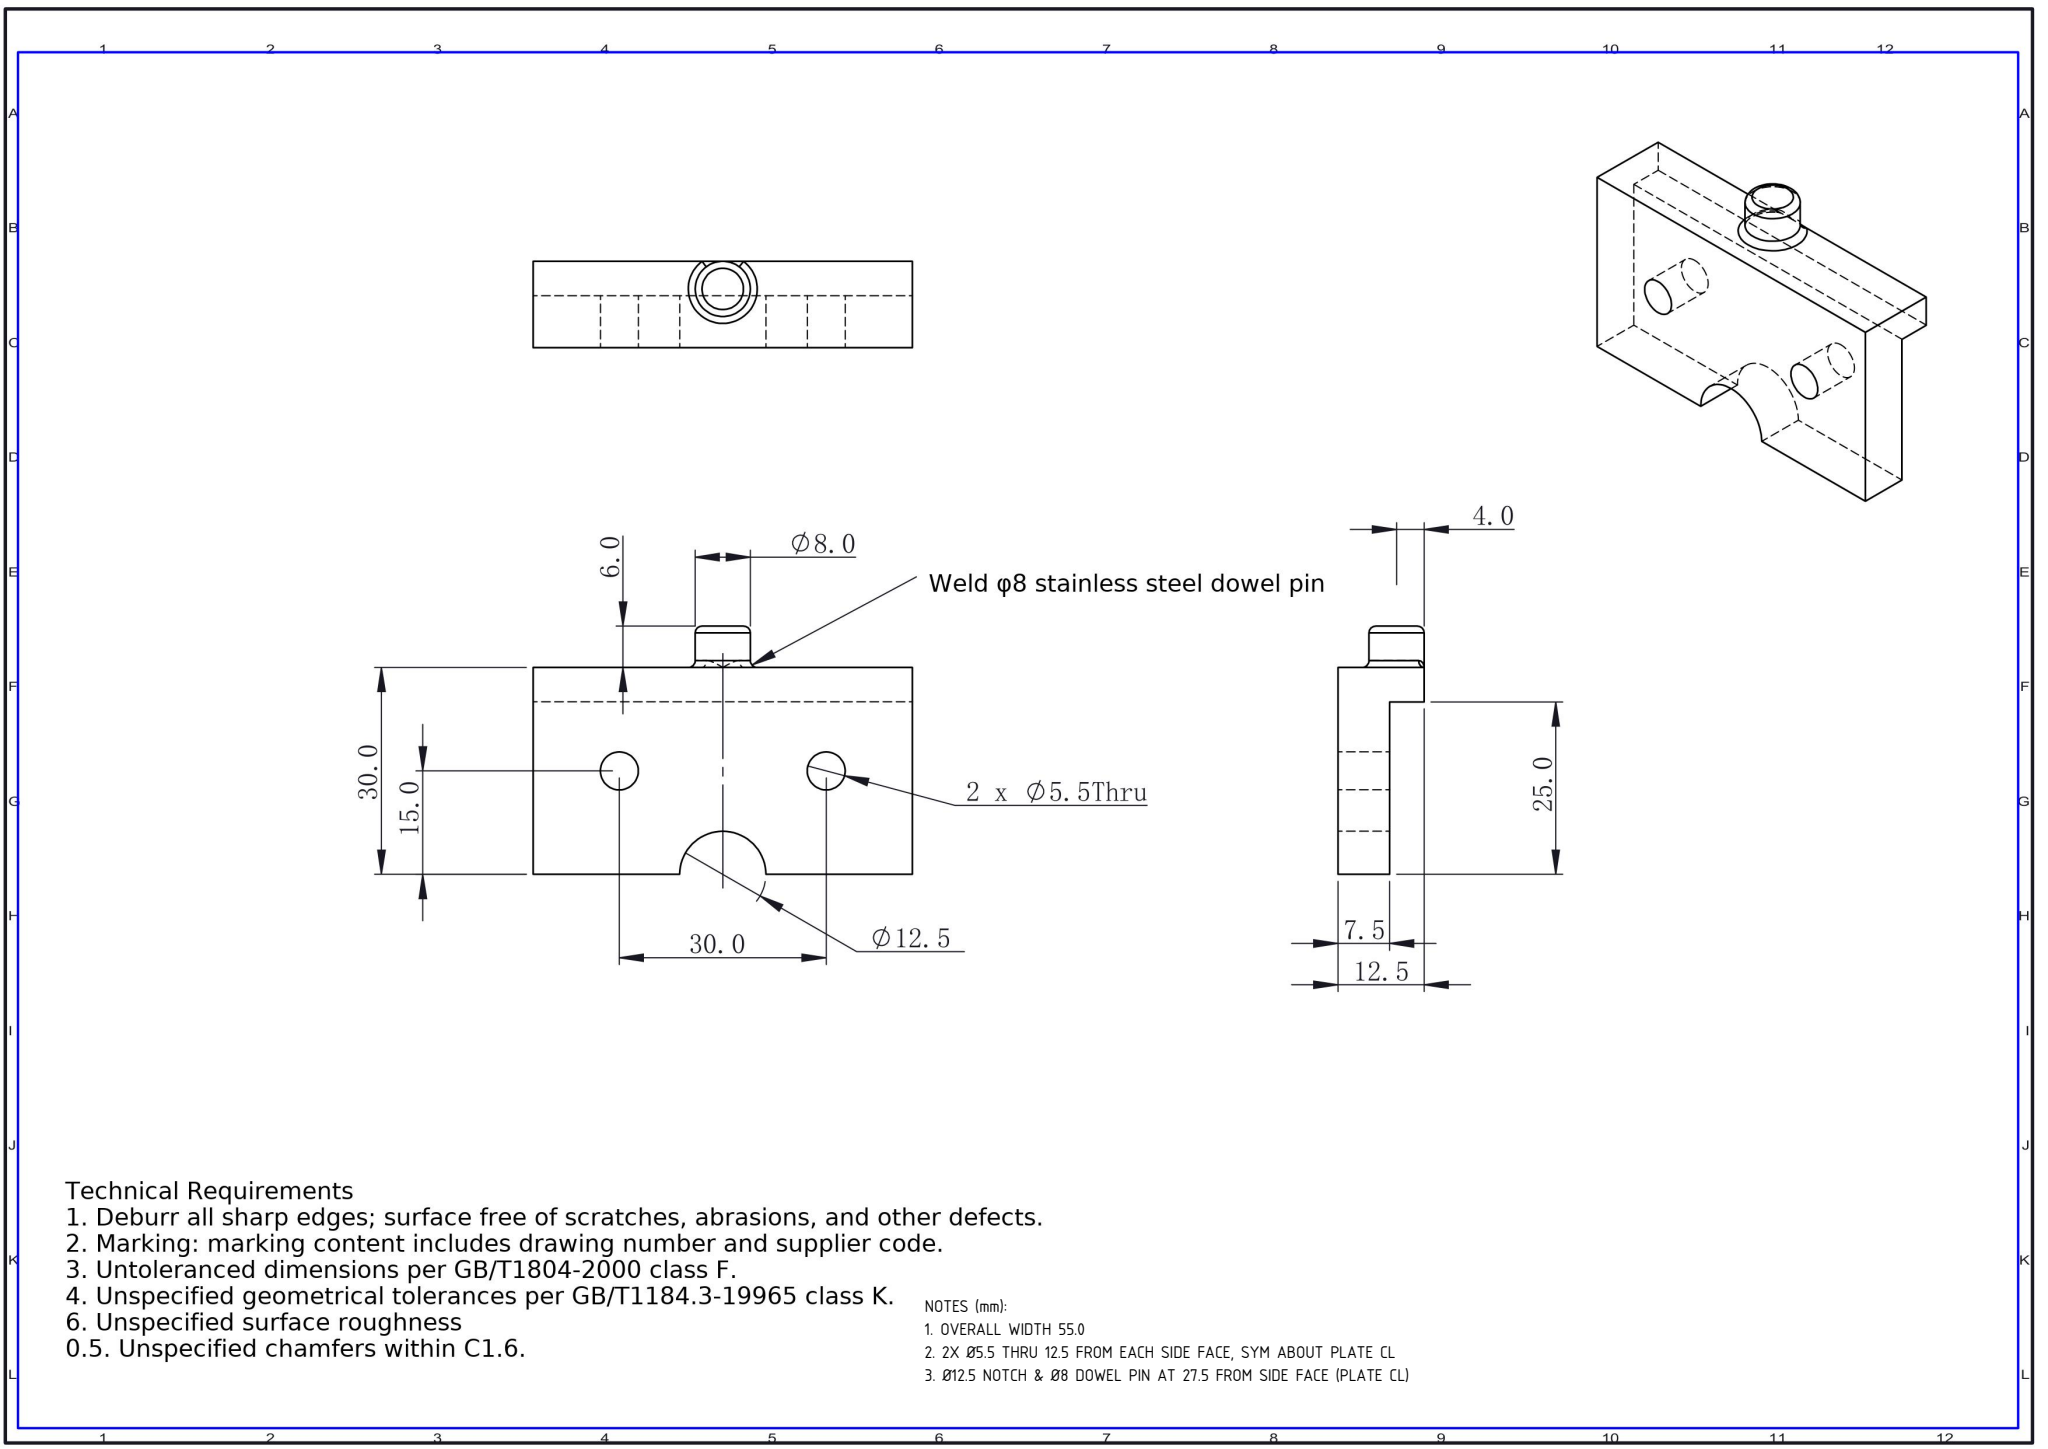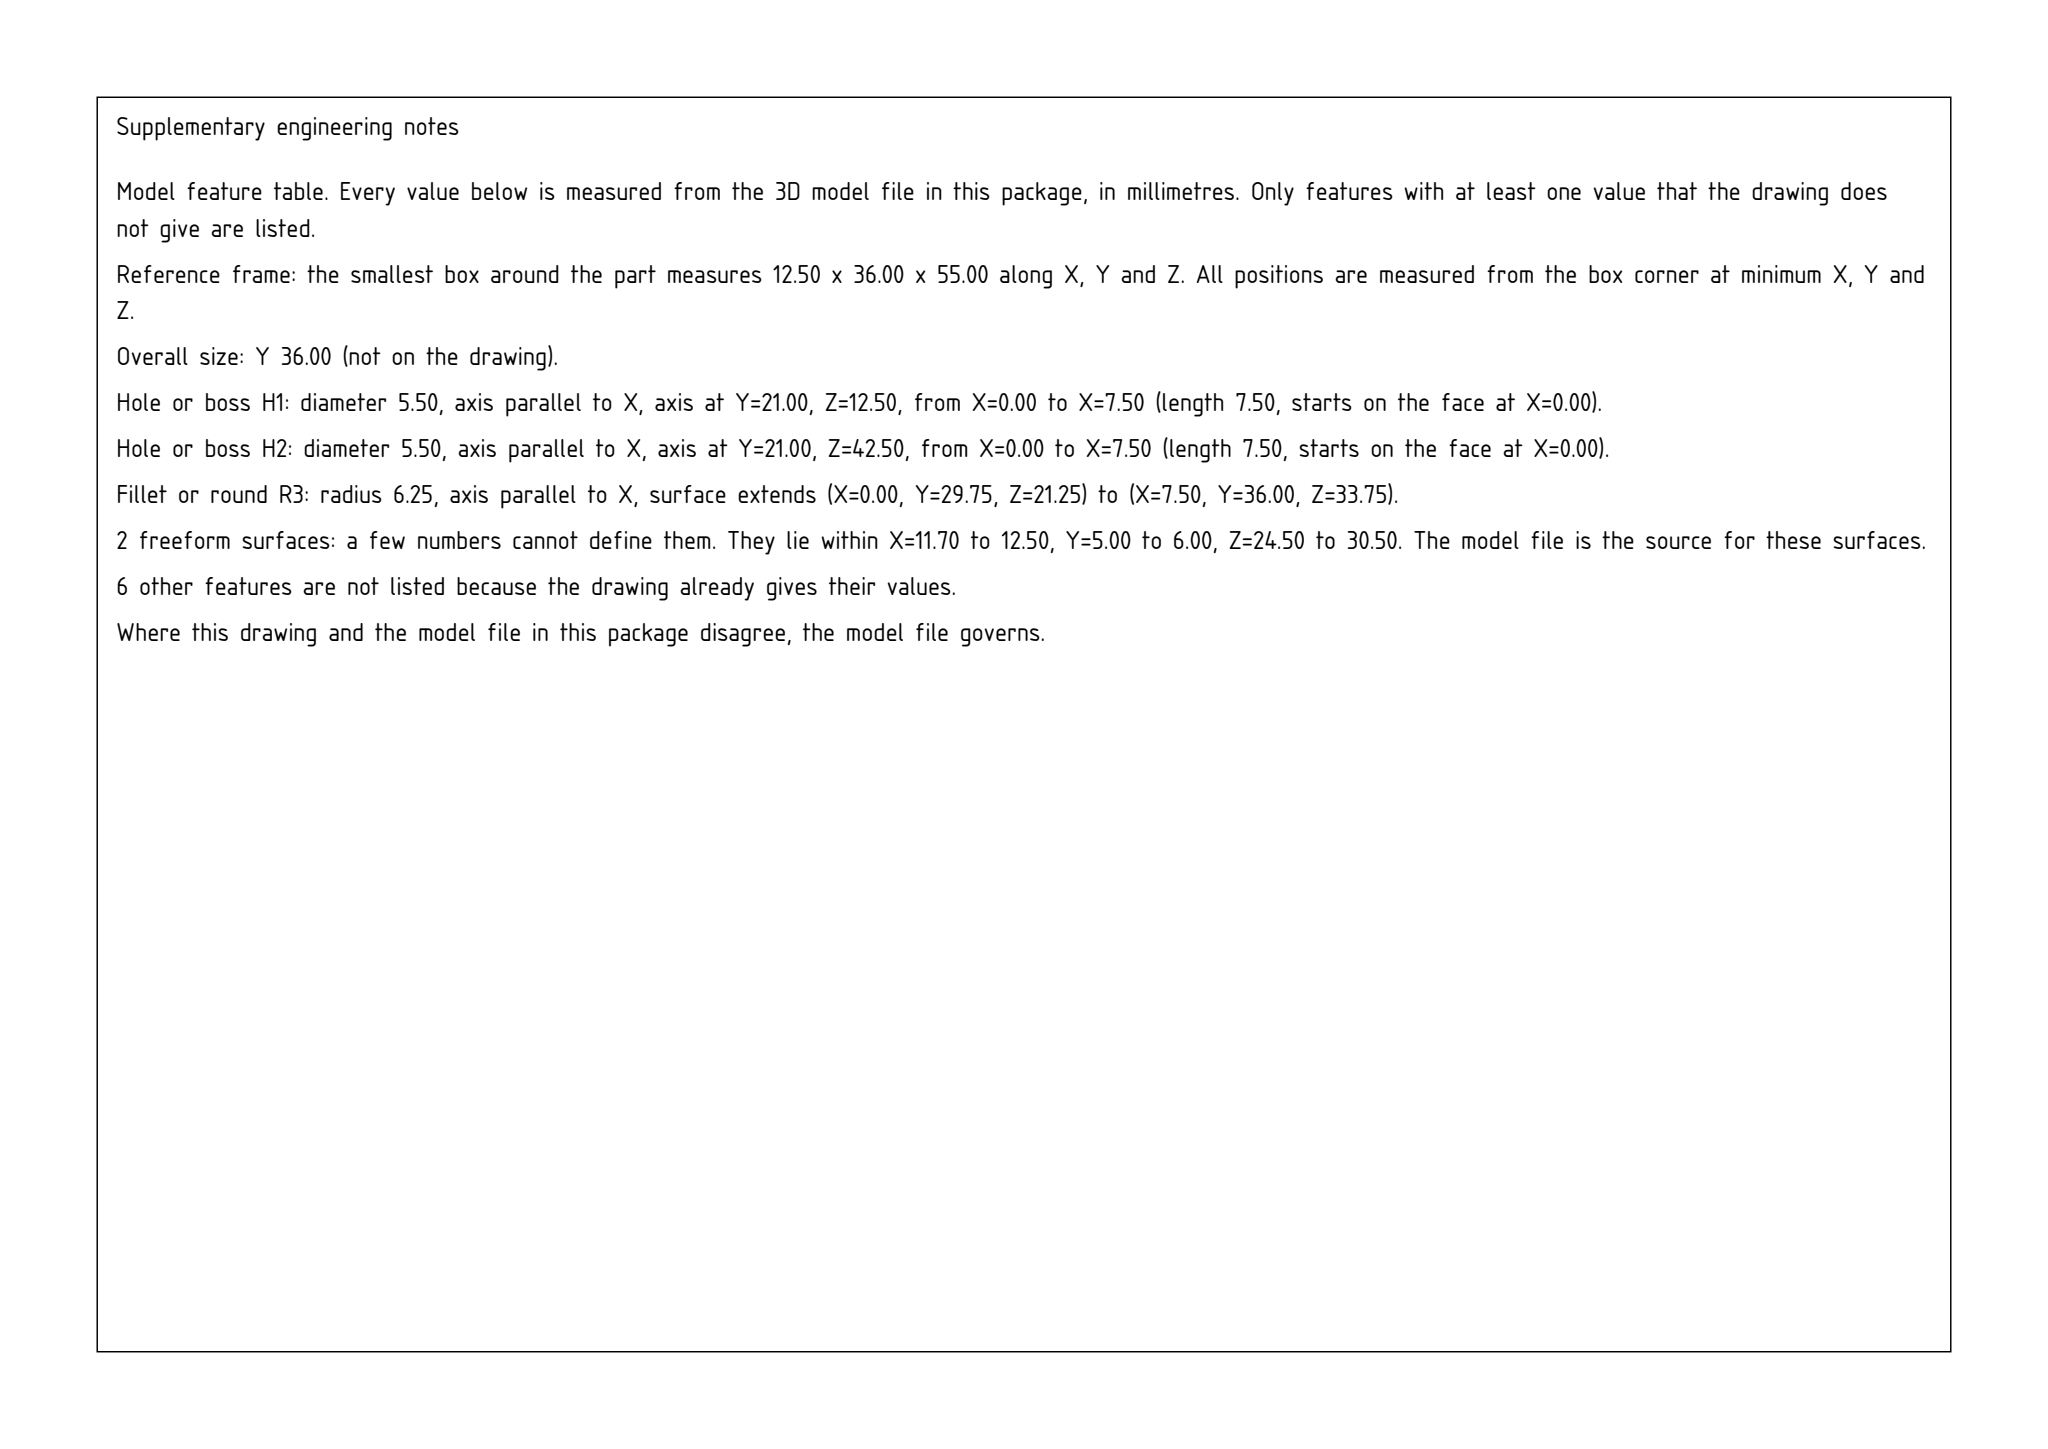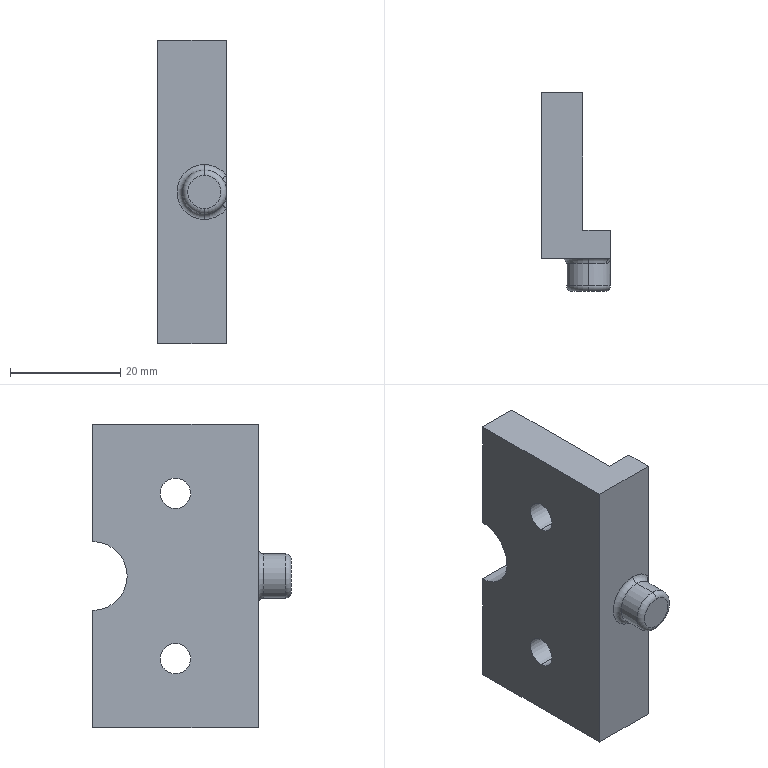Part | SolidWorks | mm | 1 solid | 25 faces | box 12.5 x 36 x 55 mm | volume 13235 mm3 | plane 10 | cylinder 8 | torus 5 | spline 2 | commonest cylinder face diameters 5.5 x4 8 x2 12.5 x2
Drawing notes:
OVERALL WIDTH 55.0 | from the solid: bbox z = 55.0 (planes z=0 and z=55)
2X Ø5.5 THRU 12.5 FROM EACH SIDE FACE, SYM ABOUT PLATE CL | from the solid: cyl Ø5.5 at z=12.5 and z=42.5, width 55.0
Ø12.5 NOTCH & Ø8 DOWEL PIN AT 27.5 FROM SIDE FACE (PLATE CL) | from the solid: Ø12.5 and Ø8 axes at z=27.5 = 55.0/2
STEP:
#1=CARTESIAN_POINT('',(8.5,-35.,31.5));
#2=VERTEX_POINT('',#1);
#3=CARTESIAN_POINT('',(8.5,-35.,23.5));
#4=VERTEX_POINT('',#3);
#5=CARTESIAN_POINT('',(8.5,-35.,27.5));
#6=DIRECTION('',(0.,1.,0.));
#7=DIRECTION('',(0.,0.,-1.));
#8=AXIS2_PLACEMENT_3D('',#5,#6,#7);
#9=CIRCLE('',#8,4.);
#10=EDGE_CURVE('',#2,#4,#9,.T.);
#11=ORIENTED_EDGE('',*,*,#10,.F.);
#12=CARTESIAN_POINT('',(8.5,-36.,30.5));
#13=VERTEX_POINT('',#12);
#14=CARTESIAN_POINT('',(8.5,-35.,30.5));
#15=DIRECTION('',(1.,0.,-0.));
#16=DIRECTION('',(0.,0.,-1.));
#17=AXIS2_PLACEMENT_3D('',#14,#15,#16);
#18=CIRCLE('',#17,1.);
#19=EDGE_CURVE('',#2,#13,#18,.T.);
#20=ORIENTED_EDGE('',*,*,#19,.T.);
#21=CARTESIAN_POINT('',(8.5,-36.,24.5));
#22=VERTEX_POINT('',#21);
#23=CARTESIAN_POINT('',(8.5,-36.,27.5));
#24=DIRECTION('',(0.,-1.,0.));
#25=DIRECTION('',(0.,0.,-1.));
#26=AXIS2_PLACEMENT_3D('',#23,#24,#25);
#27=CIRCLE('',#26,3.);
#28=EDGE_CURVE('',#22,#13,#27,.T.);
#29=ORIENTED_EDGE('',*,*,#28,.F.);
#30=CARTESIAN_POINT('',(8.5,-35.,24.5));
#31=DIRECTION('',(-1.,0.,0.));
#32=DIRECTION('',(0.,0.,1.));
#33=AXIS2_PLACEMENT_3D('',#30,#31,#32);
#34=CIRCLE('',#33,1.);
#35=EDGE_CURVE('',#4,#22,#34,.T.);
#36=ORIENTED_EDGE('',*,*,#35,.F.);
#37=EDGE_LOOP('',(#11,#20,#29,#36));
#38=FACE_OUTER_BOUND('',#37,.T.);
#39=CARTESIAN_POINT('',(8.5,-35.,27.5));
#40=DIRECTION('',(0.,-1.,0.));
#41=DIRECTION('',(0.,0.,-1.));
#42=AXIS2_PLACEMENT_3D('',#39,#40,#41);
#43=TOROIDAL_SURFACE('',#42,3.,1.);
#44=ADVANCED_FACE('',(#38),#43,.T.);
#45=CARTESIAN_POINT('',(8.5,-30.,22.5));
#46=VERTEX_POINT('',#45);
#47=CARTESIAN_POINT('',(8.5,-30.,32.5));
#48=VERTEX_POINT('',#47);
#49=CARTESIAN_POINT('',(8.5,-30.,27.5));
#50=DIRECTION('',(0.,1.,0.));
#51=DIRECTION('',(0.,0.,1.));
#52=AXIS2_PLACEMENT_3D('',#49,#50,#51);
#53=CIRCLE('',#52,5.);
#54=EDGE_CURVE('',#46,#48,#53,.T.);
#55=ORIENTED_EDGE('',*,*,#54,.F.);
#56=CARTESIAN_POINT('',(8.5,-31.,23.5));
#57=VERTEX_POINT('',#56);
#58=CARTESIAN_POINT('',(8.5,-31.,22.5));
#59=DIRECTION('',(1.,0.,0.));
#60=DIRECTION('',(0.,0.,-1.));
#61=AXIS2_PLACEMENT_3D('',#58,#59,#60);
#62=CIRCLE('',#61,1.);
#63=EDGE_CURVE('',#46,#57,#62,.T.);
#64=ORIENTED_EDGE('',*,*,#63,.T.);
#65=CARTESIAN_POINT('',(8.5,-31.,31.5));
#66=VERTEX_POINT('',#65);
#67=CARTESIAN_POINT('',(8.5,-31.,27.5));
#68=DIRECTION('',(0.,-1.,0.));
#69=DIRECTION('',(0.,0.,1.));
#70=AXIS2_PLACEMENT_3D('',#67,#68,#69);
#71=CIRCLE('',#70,4.);
#72=EDGE_CURVE('',#66,#57,#71,.T.);
#73=ORIENTED_EDGE('',*,*,#72,.F.);
#74=CARTESIAN_POINT('',(8.5,-31.,32.5));
#75=DIRECTION('',(-1.,0.,0.));
#76=DIRECTION('',(0.,0.,1.));
#77=AXIS2_PLACEMENT_3D('',#74,#75,#76);
#78=CIRCLE('',#77,1.);
#79=EDGE_CURVE('',#48,#66,#78,.T.);
#80=ORIENTED_EDGE('',*,*,#79,.F.);
#81=EDGE_LOOP('',(#55,#64,#73,#80));
#82=FACE_OUTER_BOUND('',#81,.T.);
#83=CARTESIAN_POINT('',(8.5,-31.,27.5));
#84=DIRECTION('',(0.,1.,0.));
#85=DIRECTION('',(0.,0.,1.));
#86=AXIS2_PLACEMENT_3D('',#83,#84,#85);
#87=TOROIDAL_SURFACE('',#86,5.,1.);
#88=ADVANCED_FACE('',(#82),#87,.F.);
#89=CARTESIAN_POINT('',(12.5,-30.,30.5));
#90=VERTEX_POINT('',#89);
#91=CARTESIAN_POINT('',(8.5,-30.,27.5));
#92=DIRECTION('',(0.,1.,0.));
#93=DIRECTION('',(0.,0.,1.));
#94=AXIS2_PLACEMENT_3D('',#91,#92,#93);
#95=CIRCLE('',#94,5.);
#96=EDGE_CURVE('',#48,#90,#95,.T.);
#97=ORIENTED_EDGE('',*,*,#96,.F.);
#98=ORIENTED_EDGE('',*,*,#79,.T.);
#99=CARTESIAN_POINT('',(11.7,-31.,29.9));
#100=VERTEX_POINT('',#99);
#101=CARTESIAN_POINT('',(8.5,-31.,27.5));
#102=DIRECTION('',(0.,-1.,0.));
#103=DIRECTION('',(0.,0.,1.));
#104=AXIS2_PLACEMENT_3D('',#101,#102,#103);
#105=CIRCLE('',#104,4.);
#106=EDGE_CURVE('',#100,#66,#105,.T.);
#107=ORIENTED_EDGE('',*,*,#106,.F.);
#108=CARTESIAN_POINT('',(12.5,-31.,30.5));
#109=DIRECTION('',(-0.6,0.,0.8));
#110=DIRECTION('',(0.8,0.,0.6));
#111=AXIS2_PLACEMENT_3D('',#108,#109,#110);
#112=CIRCLE('',#111,1.);
#113=EDGE_CURVE('',#90,#100,#112,.T.);
#114=ORIENTED_EDGE('',*,*,#113,.F.);
#115=EDGE_LOOP('',(#97,#98,#107,#114));
#116=FACE_OUTER_BOUND('',#115,.T.);
#117=CARTESIAN_POINT('',(8.5,-31.,27.5));
#118=DIRECTION('',(0.,1.,0.));
#119=DIRECTION('',(0.,0.,1.));
#120=AXIS2_PLACEMENT_3D('',#117,#118,#119);
#121=TOROIDAL_SURFACE('',#120,5.,1.);
#122=ADVANCED_FACE('',(#116),#121,.F.);
#123=ORIENTED_EDGE('',*,*,#10,.T.);
#124=CARTESIAN_POINT('',(8.5,-36.,23.5));
#125=DIRECTION('',(0.,1.,0.));
#126=VECTOR('',#125,1000.);
#127=LINE('',#124,#126);
#128=EDGE_CURVE('',#4,#57,#127,.T.);
#129=ORIENTED_EDGE('',*,*,#128,.T.);
#130=CARTESIAN_POINT('',(11.7,-31.,25.1));
#131=VERTEX_POINT('',#130);
#132=CARTESIAN_POINT('',(8.5,-31.,27.5));
#133=DIRECTION('',(0.,-1.,0.));
#134=DIRECTION('',(0.,0.,1.));
#135=AXIS2_PLACEMENT_3D('',#132,#133,#134);
#136=CIRCLE('',#135,4.);
#137=EDGE_CURVE('',#57,#131,#136,.T.);
#138=ORIENTED_EDGE('',*,*,#137,.T.);
#139=CARTESIAN_POINT('',(12.5,-30.,27.5));
#140=VERTEX_POINT('',#139);
#141=CARTESIAN_POINT('',(11.7,-31.,25.1));
#142=CARTESIAN_POINT('',(11.842,-31.,25.289));
#143=CARTESIAN_POINT('',(11.961,-30.956,25.482));
#144=CARTESIAN_POINT('',(12.165,-30.826,25.882));
#145=CARTESIAN_POINT('',(12.247,-30.741,26.083));
#146=CARTESIAN_POINT('',(12.375,-30.551,26.485));
#147=CARTESIAN_POINT('',(12.422,-30.447,26.686));
#148=CARTESIAN_POINT('',(12.485,-30.227,27.093));
#149=CARTESIAN_POINT('',(12.5,-30.113,27.298));
#150=CARTESIAN_POINT('',(12.5,-30.,27.5));
#151=B_SPLINE_CURVE_WITH_KNOTS('',3,(#141,#142,#143,#144,#145,#146,#147,#148,#149,#150),.UNSPECIFIED.,.F.,.F.,(4,2,2,2,4),(0.,0.0006946,0.001389,0.002084,0.002779),.UNSPECIFIED.);
#152=EDGE_CURVE('',#131,#140,#151,.T.);
#153=ORIENTED_EDGE('',*,*,#152,.T.);
#154=CARTESIAN_POINT('',(12.5,-30.,27.5));
#155=CARTESIAN_POINT('',(12.5,-30.227,27.907));
#156=CARTESIAN_POINT('',(12.439,-30.457,28.315));
#157=CARTESIAN_POINT('',(12.247,-30.741,28.917));
#158=CARTESIAN_POINT('',(12.165,-30.826,29.118));
#159=CARTESIAN_POINT('',(11.961,-30.956,29.518));
#160=CARTESIAN_POINT('',(11.842,-31.,29.711));
#161=CARTESIAN_POINT('',(11.7,-31.,29.9));
#162=B_SPLINE_CURVE_WITH_KNOTS('',3,(#154,#155,#156,#157,#158,#159,#160,#161),.UNSPECIFIED.,.F.,.F.,(4,2,2,4),(-0.00001266,0.001384,0.002083,0.002782),.UNSPECIFIED.);
#163=EDGE_CURVE('',#140,#100,#162,.T.);
#164=ORIENTED_EDGE('',*,*,#163,.T.);
#165=ORIENTED_EDGE('',*,*,#106,.T.);
#166=CARTESIAN_POINT('',(8.5,-36.,31.5));
#167=DIRECTION('',(0.,1.,0.));
#168=VECTOR('',#167,1000.);
#169=LINE('',#166,#168);
#170=EDGE_CURVE('',#2,#66,#169,.T.);
#171=ORIENTED_EDGE('',*,*,#170,.F.);
#172=EDGE_LOOP('',(#123,#129,#138,#153,#164,#165,#171));
#173=FACE_OUTER_BOUND('',#172,.T.);
#174=CARTESIAN_POINT('',(8.5,-36.,27.5));
#175=DIRECTION('',(0.,1.,0.));
#176=DIRECTION('',(0.,0.,1.));
#177=AXIS2_PLACEMENT_3D('',#174,#175,#176);
#178=CYLINDRICAL_SURFACE('',#177,4.);
#179=ADVANCED_FACE('',(#173),#178,.T.);
#180=CARTESIAN_POINT('',(7.5,-15.,9.75));
#181=VERTEX_POINT('',#180);
#182=CARTESIAN_POINT('',(7.5,-15.,15.25));
#183=VERTEX_POINT('',#182);
#184=CARTESIAN_POINT('',(7.5,-15.,12.5));
#185=DIRECTION('',(-1.,-0.,0.));
#186=DIRECTION('',(0.,-1.,0.));
#187=AXIS2_PLACEMENT_3D('',#184,#185,#186);
#188=CIRCLE('',#187,2.75);
#189=EDGE_CURVE('',#181,#183,#188,.T.);
#190=ORIENTED_EDGE('',*,*,#189,.F.);
#191=CARTESIAN_POINT('',(0.,-15.,9.75));
#192=VERTEX_POINT('',#191);
#193=CARTESIAN_POINT('',(0.,-15.,9.75));
#194=DIRECTION('',(-1.,0.,0.));
#195=VECTOR('',#194,1000.);
#196=LINE('',#193,#195);
#197=EDGE_CURVE('',#181,#192,#196,.T.);
#198=ORIENTED_EDGE('',*,*,#197,.T.);
#199=CARTESIAN_POINT('',(0.,-15.,15.25));
#200=VERTEX_POINT('',#199);
#201=CARTESIAN_POINT('',(0.,-15.,12.5));
#202=DIRECTION('',(-1.,0.,0.));
#203=DIRECTION('',(0.,0.,1.));
#204=AXIS2_PLACEMENT_3D('',#201,#202,#203);
#205=CIRCLE('',#204,2.75);
#206=EDGE_CURVE('',#192,#200,#205,.T.);
#207=ORIENTED_EDGE('',*,*,#206,.T.);
#208=CARTESIAN_POINT('',(0.,-15.,15.25));
#209=DIRECTION('',(-1.,0.,0.));
#210=VECTOR('',#209,1000.);
#211=LINE('',#208,#210);
#212=EDGE_CURVE('',#183,#200,#211,.T.);
#213=ORIENTED_EDGE('',*,*,#212,.F.);
#214=EDGE_LOOP('',(#190,#198,#207,#213));
#215=FACE_OUTER_BOUND('',#214,.T.);
#216=CARTESIAN_POINT('',(0.,-15.,12.5));
#217=DIRECTION('',(-1.,0.,0.));
#218=DIRECTION('',(0.,0.,1.));
#219=AXIS2_PLACEMENT_3D('',#216,#217,#218);
#220=CYLINDRICAL_SURFACE('',#219,2.75);
#221=ADVANCED_FACE('',(#215),#220,.F.);
#222=CARTESIAN_POINT('',(7.5,-15.,39.75));
#223=VERTEX_POINT('',#222);
#224=CARTESIAN_POINT('',(7.5,-15.,45.25));
#225=VERTEX_POINT('',#224);
#226=CARTESIAN_POINT('',(7.5,-15.,42.5));
#227=DIRECTION('',(-1.,-0.,0.));
#228=DIRECTION('',(0.,-1.,0.));
#229=AXIS2_PLACEMENT_3D('',#226,#227,#228);
#230=CIRCLE('',#229,2.75);
#231=EDGE_CURVE('',#223,#225,#230,.T.);
#232=ORIENTED_EDGE('',*,*,#231,.F.);
#233=CARTESIAN_POINT('',(0.,-15.,39.75));
#234=VERTEX_POINT('',#233);
#235=CARTESIAN_POINT('',(0.,-15.,39.75));
#236=DIRECTION('',(-1.,0.,0.));
#237=VECTOR('',#236,1000.);
#238=LINE('',#235,#237);
#239=EDGE_CURVE('',#223,#234,#238,.T.);
#240=ORIENTED_EDGE('',*,*,#239,.T.);
#241=CARTESIAN_POINT('',(0.,-15.,45.25));
#242=VERTEX_POINT('',#241);
#243=CARTESIAN_POINT('',(0.,-15.,42.5));
#244=DIRECTION('',(-1.,0.,0.));
#245=DIRECTION('',(0.,0.,1.));
#246=AXIS2_PLACEMENT_3D('',#243,#244,#245);
#247=CIRCLE('',#246,2.75);
#248=EDGE_CURVE('',#234,#242,#247,.T.);
#249=ORIENTED_EDGE('',*,*,#248,.T.);
#250=CARTESIAN_POINT('',(0.,-15.,45.25));
#251=DIRECTION('',(-1.,0.,0.));
#252=VECTOR('',#251,1000.);
#253=LINE('',#250,#252);
#254=EDGE_CURVE('',#225,#242,#253,.T.);
#255=ORIENTED_EDGE('',*,*,#254,.F.);
#256=EDGE_LOOP('',(#232,#240,#249,#255));
#257=FACE_OUTER_BOUND('',#256,.T.);
#258=CARTESIAN_POINT('',(0.,-15.,42.5));
#259=DIRECTION('',(-1.,0.,0.));
#260=DIRECTION('',(0.,0.,1.));
#261=AXIS2_PLACEMENT_3D('',#258,#259,#260);
#262=CYLINDRICAL_SURFACE('',#261,2.75);
#263=ADVANCED_FACE('',(#257),#262,.F.);
#264=CARTESIAN_POINT('',(7.5,-6.25,27.5));
#265=VERTEX_POINT('',#264);
#266=CARTESIAN_POINT('',(7.5,0.,33.75));
#267=VERTEX_POINT('',#266);
#268=CARTESIAN_POINT('',(7.5,0.,27.5));
#269=DIRECTION('',(-1.,-0.,0.));
#270=DIRECTION('',(0.,-1.,0.));
#271=AXIS2_PLACEMENT_3D('',#268,#269,#270);
#272=CIRCLE('',#271,6.25);
#273=EDGE_CURVE('',#265,#267,#272,.T.);
#274=ORIENTED_EDGE('',*,*,#273,.F.);
#275=CARTESIAN_POINT('',(0.,-6.25,27.5));
#276=VERTEX_POINT('',#275);
#277=CARTESIAN_POINT('',(12.5,-6.25,27.5));
#278=DIRECTION('',(-1.,-0.,0.));
#279=VECTOR('',#278,1000.);
#280=LINE('',#277,#279);
#281=EDGE_CURVE('',#265,#276,#280,.T.);
#282=ORIENTED_EDGE('',*,*,#281,.T.);
#283=CARTESIAN_POINT('',(0.,0.,33.75));
#284=VERTEX_POINT('',#283);
#285=CARTESIAN_POINT('',(0.,0.,27.5));
#286=DIRECTION('',(-1.,-0.,0.));
#287=DIRECTION('',(0.,-1.,0.));
#288=AXIS2_PLACEMENT_3D('',#285,#286,#287);
#289=CIRCLE('',#288,6.25);
#290=EDGE_CURVE('',#276,#284,#289,.T.);
#291=ORIENTED_EDGE('',*,*,#290,.T.);
#292=CARTESIAN_POINT('',(12.5,0.,33.75));
#293=DIRECTION('',(-1.,-0.,0.));
#294=VECTOR('',#293,1000.);
#295=LINE('',#292,#294);
#296=EDGE_CURVE('',#267,#284,#295,.T.);
#297=ORIENTED_EDGE('',*,*,#296,.F.);
#298=EDGE_LOOP('',(#274,#282,#291,#297));
#299=FACE_OUTER_BOUND('',#298,.T.);
#300=CARTESIAN_POINT('',(12.5,0.,27.5));
#301=DIRECTION('',(-1.,-0.,0.));
#302=DIRECTION('',(0.,-1.,0.));
#303=AXIS2_PLACEMENT_3D('',#300,#301,#302);
#304=CYLINDRICAL_SURFACE('',#303,6.25);
#305=ADVANCED_FACE('',(#299),#304,.F.);
#306=CARTESIAN_POINT('',(7.5,0.,55.));
#307=VERTEX_POINT('',#306);
#308=CARTESIAN_POINT('',(7.5,0.,55.));
#309=DIRECTION('',(0.,0.,-1.));
#310=VECTOR('',#309,1000.);
#311=LINE('',#308,#310);
#312=EDGE_CURVE('',#307,#267,#311,.T.);
#313=ORIENTED_EDGE('',*,*,#312,.T.);
#314=ORIENTED_EDGE('',*,*,#296,.T.);
#315=CARTESIAN_POINT('',(0.,0.,55.));
#316=VERTEX_POINT('',#315);
#317=CARTESIAN_POINT('',(0.,0.,55.));
#318=DIRECTION('',(0.,0.,-1.));
#319=VECTOR('',#318,1000.);
#320=LINE('',#317,#319);
#321=EDGE_CURVE('',#316,#284,#320,.T.);
#322=ORIENTED_EDGE('',*,*,#321,.F.);
#323=CARTESIAN_POINT('',(0.,0.,55.));
#324=DIRECTION('',(-1.,0.,0.));
#325=VECTOR('',#324,1000.);
#326=LINE('',#323,#325);
#327=EDGE_CURVE('',#307,#316,#326,.T.);
#328=ORIENTED_EDGE('',*,*,#327,.F.);
#329=EDGE_LOOP('',(#313,#314,#322,#328));
#330=FACE_OUTER_BOUND('',#329,.T.);
#331=CARTESIAN_POINT('',(0.,0.,55.));
#332=DIRECTION('',(0.,-1.,0.));
#333=DIRECTION('',(0.,0.,-1.));
#334=AXIS2_PLACEMENT_3D('',#331,#332,#333);
#335=PLANE('',#334);
#336=ADVANCED_FACE('',(#330),#335,.F.);
#337=CARTESIAN_POINT('',(0.,-15.,12.5));
#338=DIRECTION('',(-1.,0.,0.));
#339=DIRECTION('',(0.,0.,1.));
#340=AXIS2_PLACEMENT_3D('',#337,#338,#339);
#341=CIRCLE('',#340,2.75);
#342=EDGE_CURVE('',#200,#192,#341,.T.);
#343=ORIENTED_EDGE('',*,*,#342,.F.);
#344=ORIENTED_EDGE('',*,*,#206,.F.);
#345=EDGE_LOOP('',(#343,#344));
#346=FACE_BOUND('',#345,.T.);
#347=CARTESIAN_POINT('',(0.,-15.,42.5));
#348=DIRECTION('',(-1.,0.,0.));
#349=DIRECTION('',(0.,0.,1.));
#350=AXIS2_PLACEMENT_3D('',#347,#348,#349);
#351=CIRCLE('',#350,2.75);
#352=EDGE_CURVE('',#242,#234,#351,.T.);
#353=ORIENTED_EDGE('',*,*,#352,.F.);
#354=ORIENTED_EDGE('',*,*,#248,.F.);
#355=EDGE_LOOP('',(#353,#354));
#356=FACE_BOUND('',#355,.T.);
#357=ORIENTED_EDGE('',*,*,#321,.T.);
#358=ORIENTED_EDGE('',*,*,#290,.F.);
#359=CARTESIAN_POINT('',(0.,0.,21.25));
#360=VERTEX_POINT('',#359);
#361=CARTESIAN_POINT('',(0.,0.,27.5));
#362=DIRECTION('',(-1.,-0.,0.));
#363=DIRECTION('',(0.,-1.,0.));
#364=AXIS2_PLACEMENT_3D('',#361,#362,#363);
#365=CIRCLE('',#364,6.25);
#366=EDGE_CURVE('',#360,#276,#365,.T.);
#367=ORIENTED_EDGE('',*,*,#366,.F.);
#368=CARTESIAN_POINT('',(0.,0.,0.));
#369=VERTEX_POINT('',#368);
#370=CARTESIAN_POINT('',(0.,0.,55.));
#371=DIRECTION('',(0.,0.,-1.));
#372=VECTOR('',#371,1000.);
#373=LINE('',#370,#372);
#374=EDGE_CURVE('',#360,#369,#373,.T.);
#375=ORIENTED_EDGE('',*,*,#374,.T.);
#376=CARTESIAN_POINT('',(0.,-30.,0.));
#377=VERTEX_POINT('',#376);
#378=CARTESIAN_POINT('',(0.,0.,0.));
#379=DIRECTION('',(0.,-1.,0.));
#380=VECTOR('',#379,1000.);
#381=LINE('',#378,#380);
#382=EDGE_CURVE('',#369,#377,#381,.T.);
#383=ORIENTED_EDGE('',*,*,#382,.T.);
#384=CARTESIAN_POINT('',(0.,-30.,55.));
#385=VERTEX_POINT('',#384);
#386=CARTESIAN_POINT('',(0.,-30.,55.));
#387=DIRECTION('',(0.,0.,-1.));
#388=VECTOR('',#387,1000.);
#389=LINE('',#386,#388);
#390=EDGE_CURVE('',#385,#377,#389,.T.);
#391=ORIENTED_EDGE('',*,*,#390,.F.);
#392=CARTESIAN_POINT('',(0.,0.,55.));
#393=DIRECTION('',(0.,-1.,0.));
#394=VECTOR('',#393,1000.);
#395=LINE('',#392,#394);
#396=EDGE_CURVE('',#316,#385,#395,.T.);
#397=ORIENTED_EDGE('',*,*,#396,.F.);
#398=EDGE_LOOP('',(#357,#358,#367,#375,#383,#391,#397));
#399=FACE_OUTER_BOUND('',#398,.T.);
#400=CARTESIAN_POINT('',(0.,0.,55.));
#401=DIRECTION('',(1.,0.,0.));
#402=DIRECTION('',(-0.,1.,0.));
#403=AXIS2_PLACEMENT_3D('',#400,#401,#402);
#404=PLANE('',#403);
#405=ADVANCED_FACE('',(#346,#356,#399),#404,.F.);
#406=CARTESIAN_POINT('',(12.5,-30.,24.5));
#407=VERTEX_POINT('',#406);
#408=CARTESIAN_POINT('',(12.5,-30.,0.));
#409=VERTEX_POINT('',#408);
#410=CARTESIAN_POINT('',(12.5,-30.,55.));
#411=DIRECTION('',(0.,0.,-1.));
#412=VECTOR('',#411,1000.);
#413=LINE('',#410,#412);
#414=EDGE_CURVE('',#407,#409,#413,.T.);
#415=ORIENTED_EDGE('',*,*,#414,.F.);
#416=CARTESIAN_POINT('',(8.5,-30.,27.5));
#417=DIRECTION('',(0.,1.,0.));
#418=DIRECTION('',(0.,0.,1.));
#419=AXIS2_PLACEMENT_3D('',#416,#417,#418);
#420=CIRCLE('',#419,5.);
#421=EDGE_CURVE('',#407,#46,#420,.T.);
#422=ORIENTED_EDGE('',*,*,#421,.T.);
#423=ORIENTED_EDGE('',*,*,#54,.T.);
#424=ORIENTED_EDGE('',*,*,#96,.T.);
#425=CARTESIAN_POINT('',(12.5,-30.,55.));
#426=VERTEX_POINT('',#425);
#427=CARTESIAN_POINT('',(12.5,-30.,55.));
#428=DIRECTION('',(0.,0.,-1.));
#429=VECTOR('',#428,1000.);
#430=LINE('',#427,#429);
#431=EDGE_CURVE('',#426,#90,#430,.T.);
#432=ORIENTED_EDGE('',*,*,#431,.F.);
#433=CARTESIAN_POINT('',(0.,-30.,55.));
#434=DIRECTION('',(1.,0.,0.));
#435=VECTOR('',#434,1000.);
#436=LINE('',#433,#435);
#437=EDGE_CURVE('',#385,#426,#436,.T.);
#438=ORIENTED_EDGE('',*,*,#437,.F.);
#439=ORIENTED_EDGE('',*,*,#390,.T.);
#440=CARTESIAN_POINT('',(0.,-30.,0.));
#441=DIRECTION('',(1.,0.,0.));
#442=VECTOR('',#441,1000.);
#443=LINE('',#440,#442);
#444=EDGE_CURVE('',#377,#409,#443,.T.);
#445=ORIENTED_EDGE('',*,*,#444,.T.);
#446=EDGE_LOOP('',(#415,#422,#423,#424,#432,#438,#439,#445));
#447=FACE_OUTER_BOUND('',#446,.T.);
#448=CARTESIAN_POINT('',(0.,-30.,55.));
#449=DIRECTION('',(0.,1.,0.));
#450=DIRECTION('',(0.,0.,1.));
#451=AXIS2_PLACEMENT_3D('',#448,#449,#450);
#452=PLANE('',#451);
#453=ADVANCED_FACE('',(#447),#452,.F.);
#454=CARTESIAN_POINT('',(12.5,-25.,0.));
#455=VERTEX_POINT('',#454);
#456=CARTESIAN_POINT('',(12.5,-25.,0.));
#457=DIRECTION('',(0.,1.,0.));
#458=VECTOR('',#457,1000.);
#459=LINE('',#456,#458);
#460=EDGE_CURVE('',#409,#455,#459,.T.);
#461=ORIENTED_EDGE('',*,*,#460,.T.);
#462=CARTESIAN_POINT('',(12.5,-25.,55.));
#463=VERTEX_POINT('',#462);
#464=CARTESIAN_POINT('',(12.5,-25.,55.));
#465=DIRECTION('',(0.,0.,-1.));
#466=VECTOR('',#465,1000.);
#467=LINE('',#464,#466);
#468=EDGE_CURVE('',#463,#455,#467,.T.);
#469=ORIENTED_EDGE('',*,*,#468,.F.);
#470=CARTESIAN_POINT('',(12.5,-25.,55.));
#471=DIRECTION('',(0.,1.,0.));
#472=VECTOR('',#471,1000.);
#473=LINE('',#470,#472);
#474=EDGE_CURVE('',#426,#463,#473,.T.);
#475=ORIENTED_EDGE('',*,*,#474,.F.);
#476=ORIENTED_EDGE('',*,*,#431,.T.);
#477=CARTESIAN_POINT('',(12.5,-30.,55.));
#478=DIRECTION('',(0.,0.,-1.));
#479=VECTOR('',#478,1000.);
#480=LINE('',#477,#479);
#481=EDGE_CURVE('',#90,#140,#480,.T.);
#482=ORIENTED_EDGE('',*,*,#481,.T.);
#483=CARTESIAN_POINT('',(12.5,-30.,55.));
#484=DIRECTION('',(0.,0.,-1.));
#485=VECTOR('',#484,1000.);
#486=LINE('',#483,#485);
#487=EDGE_CURVE('',#140,#407,#486,.T.);
#488=ORIENTED_EDGE('',*,*,#487,.T.);
#489=ORIENTED_EDGE('',*,*,#414,.T.);
#490=EDGE_LOOP('',(#461,#469,#475,#476,#482,#488,#489));
#491=FACE_OUTER_BOUND('',#490,.T.);
#492=CARTESIAN_POINT('',(12.5,-25.,55.));
#493=DIRECTION('',(-1.,0.,0.));
#494=DIRECTION('',(0.,0.,1.));
#495=AXIS2_PLACEMENT_3D('',#492,#493,#494);
#496=PLANE('',#495);
#497=ADVANCED_FACE('',(#491),#496,.F.);
#498=CARTESIAN_POINT('',(7.5,-25.,0.));
#499=VERTEX_POINT('',#498);
#500=CARTESIAN_POINT('',(12.5,-25.,0.));
#501=DIRECTION('',(-1.,0.,0.));
#502=VECTOR('',#501,1000.);
#503=LINE('',#500,#502);
#504=EDGE_CURVE('',#455,#499,#503,.T.);
#505=ORIENTED_EDGE('',*,*,#504,.T.);
#506=CARTESIAN_POINT('',(7.5,-25.,55.));
#507=VERTEX_POINT('',#506);
#508=CARTESIAN_POINT('',(7.5,-25.,55.));
#509=DIRECTION('',(0.,0.,-1.));
#510=VECTOR('',#509,1000.);
#511=LINE('',#508,#510);
#512=EDGE_CURVE('',#507,#499,#511,.T.);
#513=ORIENTED_EDGE('',*,*,#512,.F.);
#514=CARTESIAN_POINT('',(12.5,-25.,55.));
#515=DIRECTION('',(-1.,0.,0.));
#516=VECTOR('',#515,1000.);
#517=LINE('',#514,#516);
#518=EDGE_CURVE('',#463,#507,#517,.T.);
#519=ORIENTED_EDGE('',*,*,#518,.F.);
#520=ORIENTED_EDGE('',*,*,#468,.T.);
#521=EDGE_LOOP('',(#505,#513,#519,#520));
#522=FACE_OUTER_BOUND('',#521,.T.);
#523=CARTESIAN_POINT('',(12.5,-25.,55.));
#524=DIRECTION('',(0.,-1.,0.));
#525=DIRECTION('',(0.,0.,-1.));
#526=AXIS2_PLACEMENT_3D('',#523,#524,#525);
#527=PLANE('',#526);
#528=ADVANCED_FACE('',(#522),#527,.F.);
#529=CARTESIAN_POINT('',(7.5,-15.,12.5));
#530=DIRECTION('',(-1.,-0.,0.));
#531=DIRECTION('',(0.,-1.,0.));
#532=AXIS2_PLACEMENT_3D('',#529,#530,#531);
#533=CIRCLE('',#532,2.75);
#534=EDGE_CURVE('',#183,#181,#533,.T.);
#535=ORIENTED_EDGE('',*,*,#534,.T.);
#536=ORIENTED_EDGE('',*,*,#189,.T.);
#537=EDGE_LOOP('',(#535,#536));
#538=FACE_BOUND('',#537,.T.);
#539=CARTESIAN_POINT('',(7.5,-15.,42.5));
#540=DIRECTION('',(-1.,-0.,0.));
#541=DIRECTION('',(0.,-1.,0.));
#542=AXIS2_PLACEMENT_3D('',#539,#540,#541);
#543=CIRCLE('',#542,2.75);
#544=EDGE_CURVE('',#225,#223,#543,.T.);
#545=ORIENTED_EDGE('',*,*,#544,.T.);
#546=ORIENTED_EDGE('',*,*,#231,.T.);
#547=EDGE_LOOP('',(#545,#546));
#548=FACE_BOUND('',#547,.T.);
#549=CARTESIAN_POINT('',(7.5,0.,21.25));
#550=VERTEX_POINT('',#549);
#551=CARTESIAN_POINT('',(7.5,0.,0.));
#552=VERTEX_POINT('',#551);
#553=CARTESIAN_POINT('',(7.5,0.,55.));
#554=DIRECTION('',(0.,0.,-1.));
#555=VECTOR('',#554,1000.);
#556=LINE('',#553,#555);
#557=EDGE_CURVE('',#550,#552,#556,.T.);
#558=ORIENTED_EDGE('',*,*,#557,.F.);
#559=CARTESIAN_POINT('',(7.5,0.,27.5));
#560=DIRECTION('',(-1.,-0.,0.));
#561=DIRECTION('',(0.,-1.,0.));
#562=AXIS2_PLACEMENT_3D('',#559,#560,#561);
#563=CIRCLE('',#562,6.25);
#564=EDGE_CURVE('',#550,#265,#563,.T.);
#565=ORIENTED_EDGE('',*,*,#564,.T.);
#566=ORIENTED_EDGE('',*,*,#273,.T.);
#567=ORIENTED_EDGE('',*,*,#312,.F.);
#568=CARTESIAN_POINT('',(7.5,0.,55.));
#569=DIRECTION('',(-0.,1.,0.));
#570=VECTOR('',#569,1000.);
#571=LINE('',#568,#570);
#572=EDGE_CURVE('',#507,#307,#571,.T.);
#573=ORIENTED_EDGE('',*,*,#572,.F.);
#574=ORIENTED_EDGE('',*,*,#512,.T.);
#575=CARTESIAN_POINT('',(7.5,0.,0.));
#576=DIRECTION('',(-0.,1.,0.));
#577=VECTOR('',#576,1000.);
#578=LINE('',#575,#577);
#579=EDGE_CURVE('',#499,#552,#578,.T.);
#580=ORIENTED_EDGE('',*,*,#579,.T.);
#581=EDGE_LOOP('',(#558,#565,#566,#567,#573,#574,#580));
#582=FACE_OUTER_BOUND('',#581,.T.);
#583=CARTESIAN_POINT('',(7.5,0.,55.));
#584=DIRECTION('',(-1.,-0.,0.));
#585=DIRECTION('',(0.,-1.,0.));
#586=AXIS2_PLACEMENT_3D('',#583,#584,#585);
#587=PLANE('',#586);
#588=ADVANCED_FACE('',(#538,#548,#582),#587,.F.);
#589=ORIENTED_EDGE('',*,*,#374,.F.);
#590=CARTESIAN_POINT('',(12.5,0.,21.25));
#591=DIRECTION('',(1.,0.,0.));
#592=VECTOR('',#591,1000.);
#593=LINE('',#590,#592);
#594=EDGE_CURVE('',#360,#550,#593,.T.);
#595=ORIENTED_EDGE('',*,*,#594,.T.);
#596=ORIENTED_EDGE('',*,*,#557,.T.);
#597=CARTESIAN_POINT('',(0.,0.,0.));
#598=DIRECTION('',(-1.,0.,0.));
#599=VECTOR('',#598,1000.);
#600=LINE('',#597,#599);
#601=EDGE_CURVE('',#552,#369,#600,.T.);
#602=ORIENTED_EDGE('',*,*,#601,.T.);
#603=EDGE_LOOP('',(#589,#595,#596,#602));
#604=FACE_OUTER_BOUND('',#603,.T.);
#605=CARTESIAN_POINT('',(0.,0.,55.));
#606=DIRECTION('',(0.,-1.,0.));
#607=DIRECTION('',(0.,0.,-1.));
#608=AXIS2_PLACEMENT_3D('',#605,#606,#607);
#609=PLANE('',#608);
#610=ADVANCED_FACE('',(#604),#609,.F.);
#611=ORIENTED_EDGE('',*,*,#396,.T.);
#612=ORIENTED_EDGE('',*,*,#437,.T.);
#613=ORIENTED_EDGE('',*,*,#474,.T.);
#614=ORIENTED_EDGE('',*,*,#518,.T.);
#615=ORIENTED_EDGE('',*,*,#572,.T.);
#616=ORIENTED_EDGE('',*,*,#327,.T.);
#617=EDGE_LOOP('',(#611,#612,#613,#614,#615,#616));
#618=FACE_OUTER_BOUND('',#617,.T.);
#619=CARTESIAN_POINT('',(0.,0.,55.));
#620=DIRECTION('',(0.,0.,1.));
#621=DIRECTION('',(1.,0.,0.));
#622=AXIS2_PLACEMENT_3D('',#619,#620,#621);
#623=PLANE('',#622);
#624=ADVANCED_FACE('',(#618),#623,.T.);
#625=ORIENTED_EDGE('',*,*,#382,.F.);
#626=ORIENTED_EDGE('',*,*,#601,.F.);
#627=ORIENTED_EDGE('',*,*,#579,.F.);
#628=ORIENTED_EDGE('',*,*,#504,.F.);
#629=ORIENTED_EDGE('',*,*,#460,.F.);
#630=ORIENTED_EDGE('',*,*,#444,.F.);
#631=EDGE_LOOP('',(#625,#626,#627,#628,#629,#630));
#632=FACE_OUTER_BOUND('',#631,.T.);
#633=CARTESIAN_POINT('',(0.,0.,0.));
#634=DIRECTION('',(0.,0.,1.));
#635=DIRECTION('',(1.,0.,0.));
#636=AXIS2_PLACEMENT_3D('',#633,#634,#635);
#637=PLANE('',#636);
#638=ADVANCED_FACE('',(#632),#637,.F.);
#639=ORIENTED_EDGE('',*,*,#281,.F.);
#640=ORIENTED_EDGE('',*,*,#564,.F.);
#641=ORIENTED_EDGE('',*,*,#594,.F.);
#642=ORIENTED_EDGE('',*,*,#366,.T.);
#643=EDGE_LOOP('',(#639,#640,#641,#642));
#644=FACE_OUTER_BOUND('',#643,.T.);
#645=CARTESIAN_POINT('',(12.5,0.,27.5));
#646=DIRECTION('',(-1.,-0.,0.));
#647=DIRECTION('',(0.,-1.,0.));
#648=AXIS2_PLACEMENT_3D('',#645,#646,#647);
#649=CYLINDRICAL_SURFACE('',#648,6.25);
#650=ADVANCED_FACE('',(#644),#649,.F.);
#651=ORIENTED_EDGE('',*,*,#239,.F.);
#652=ORIENTED_EDGE('',*,*,#544,.F.);
#653=ORIENTED_EDGE('',*,*,#254,.T.);
#654=ORIENTED_EDGE('',*,*,#352,.T.);
#655=EDGE_LOOP('',(#651,#652,#653,#654));
#656=FACE_OUTER_BOUND('',#655,.T.);
#657=CARTESIAN_POINT('',(0.,-15.,42.5));
#658=DIRECTION('',(-1.,0.,0.));
#659=DIRECTION('',(0.,0.,1.));
#660=AXIS2_PLACEMENT_3D('',#657,#658,#659);
#661=CYLINDRICAL_SURFACE('',#660,2.75);
#662=ADVANCED_FACE('',(#656),#661,.F.);
#663=ORIENTED_EDGE('',*,*,#197,.F.);
#664=ORIENTED_EDGE('',*,*,#534,.F.);
#665=ORIENTED_EDGE('',*,*,#212,.T.);
#666=ORIENTED_EDGE('',*,*,#342,.T.);
#667=EDGE_LOOP('',(#663,#664,#665,#666));
#668=FACE_OUTER_BOUND('',#667,.T.);
#669=CARTESIAN_POINT('',(0.,-15.,12.5));
#670=DIRECTION('',(-1.,0.,0.));
#671=DIRECTION('',(0.,0.,1.));
#672=AXIS2_PLACEMENT_3D('',#669,#670,#671);
#673=CYLINDRICAL_SURFACE('',#672,2.75);
#674=ADVANCED_FACE('',(#668),#673,.F.);
#675=ORIENTED_EDGE('',*,*,#128,.F.);
#676=CARTESIAN_POINT('',(8.5,-35.,27.5));
#677=DIRECTION('',(0.,1.,0.));
#678=DIRECTION('',(0.,0.,-1.));
#679=AXIS2_PLACEMENT_3D('',#676,#677,#678);
#680=CIRCLE('',#679,4.);
#681=EDGE_CURVE('',#4,#2,#680,.T.);
#682=ORIENTED_EDGE('',*,*,#681,.T.);
#683=ORIENTED_EDGE('',*,*,#170,.T.);
#684=ORIENTED_EDGE('',*,*,#72,.T.);
#685=EDGE_LOOP('',(#675,#682,#683,#684));
#686=FACE_OUTER_BOUND('',#685,.T.);
#687=CARTESIAN_POINT('',(8.5,-36.,27.5));
#688=DIRECTION('',(0.,1.,0.));
#689=DIRECTION('',(0.,0.,1.));
#690=AXIS2_PLACEMENT_3D('',#687,#688,#689);
#691=CYLINDRICAL_SURFACE('',#690,4.);
#692=ADVANCED_FACE('',(#686),#691,.T.);
#693=ORIENTED_EDGE('',*,*,#28,.T.);
#694=CARTESIAN_POINT('',(8.5,-36.,27.5));
#695=DIRECTION('',(0.,-1.,0.));
#696=DIRECTION('',(0.,0.,-1.));
#697=AXIS2_PLACEMENT_3D('',#694,#695,#696);
#698=CIRCLE('',#697,3.);
#699=EDGE_CURVE('',#13,#22,#698,.T.);
#700=ORIENTED_EDGE('',*,*,#699,.T.);
#701=EDGE_LOOP('',(#693,#700));
#702=FACE_OUTER_BOUND('',#701,.T.);
#703=CARTESIAN_POINT('',(8.5,-36.,27.5));
#704=DIRECTION('',(0.,-1.,0.));
#705=DIRECTION('',(0.,0.,-1.));
#706=AXIS2_PLACEMENT_3D('',#703,#704,#705);
#707=PLANE('',#706);
#708=ADVANCED_FACE('',(#702),#707,.T.);
#709=ORIENTED_EDGE('',*,*,#487,.F.);
#710=ORIENTED_EDGE('',*,*,#152,.F.);
#711=CARTESIAN_POINT('',(12.5,-31.,24.5));
#712=DIRECTION('',(0.6,0.,0.8));
#713=DIRECTION('',(-0.8,-0.,0.6));
#714=AXIS2_PLACEMENT_3D('',#711,#712,#713);
#715=CIRCLE('',#714,1.);
#716=EDGE_CURVE('',#407,#131,#715,.T.);
#717=ORIENTED_EDGE('',*,*,#716,.F.);
#718=EDGE_LOOP('',(#709,#710,#717));
#719=FACE_OUTER_BOUND('',#718,.T.);
#720=CARTESIAN_POINT('',(11.7,-31.,25.1));
#721=CARTESIAN_POINT('',(11.7,-30.,25.1));
#722=CARTESIAN_POINT('',(12.5,-30.,24.5));
#723=CARTESIAN_POINT('',(11.837,-31.,25.283));
#724=CARTESIAN_POINT('',(11.771,-30.13,25.195));
#725=CARTESIAN_POINT('',(12.5,-30.,24.729));
#726=CARTESIAN_POINT('',(11.955,-30.958,25.472));
#727=CARTESIAN_POINT('',(11.882,-30.213,25.349));
#728=CARTESIAN_POINT('',(12.5,-30.,24.966));
#729=CARTESIAN_POINT('',(12.158,-30.832,25.866));
#730=CARTESIAN_POINT('',(12.088,-30.291,25.713));
#731=CARTESIAN_POINT('',(12.5,-30.,25.458));
#732=CARTESIAN_POINT('',(12.24,-30.748,26.067));
#733=CARTESIAN_POINT('',(12.185,-30.294,25.92));
#734=CARTESIAN_POINT('',(12.5,-30.,25.709));
#735=CARTESIAN_POINT('',(12.436,-30.465,26.671));
#736=CARTESIAN_POINT('',(12.409,-30.236,26.544));
#737=CARTESIAN_POINT('',(12.5,-30.,26.464));
#738=CARTESIAN_POINT('',(12.5,-30.231,27.086));
#739=CARTESIAN_POINT('',(12.5,-30.116,27.035));
#740=CARTESIAN_POINT('',(12.5,-30.,26.982));
#741=CARTESIAN_POINT('',(12.5,-30.,27.5));
#742=CARTESIAN_POINT('',(12.5,-30.,27.5));
#743=CARTESIAN_POINT('',(12.5,-30.,27.5));
#744=(BOUNDED_SURFACE()B_SPLINE_SURFACE(3,2,((#720,#721,#722),(#723,#724,#725),(#726,#727,#728),(#729,#730,#731),(#732,#733,#734),(#735,#736,#737),(#738,#739,#740),(#741,#742,#743)),.UNSPECIFIED.,.F.,.F.,.T.)B_SPLINE_SURFACE_WITH_KNOTS((4,2,2,4),(3,3),(0.001927,0.002779,0.003632,0.005338),(0.,1.),.UNSPECIFIED.)GEOMETRIC_REPRESENTATION_ITEM()RATIONAL_B_SPLINE_SURFACE(((1.,0.7071,1.),(1.,0.7556,1.),(1.,0.7984,1.),(1.,0.8726,1.),(1.,0.9032,1.),(1.,0.9759,1.),(1.,1.,1.),(1.,1.,1.)))REPRESENTATION_ITEM('')SURFACE());
#745=ADVANCED_FACE('',(#719),#744,.F.);
#746=ORIENTED_EDGE('',*,*,#63,.F.);
#747=ORIENTED_EDGE('',*,*,#421,.F.);
#748=ORIENTED_EDGE('',*,*,#716,.T.);
#749=ORIENTED_EDGE('',*,*,#137,.F.);
#750=EDGE_LOOP('',(#746,#747,#748,#749));
#751=FACE_OUTER_BOUND('',#750,.T.);
#752=CARTESIAN_POINT('',(8.5,-31.,27.5));
#753=DIRECTION('',(0.,1.,0.));
#754=DIRECTION('',(0.,0.,1.));
#755=AXIS2_PLACEMENT_3D('',#752,#753,#754);
#756=TOROIDAL_SURFACE('',#755,5.,1.);
#757=ADVANCED_FACE('',(#751),#756,.F.);
#758=ORIENTED_EDGE('',*,*,#163,.F.);
#759=ORIENTED_EDGE('',*,*,#481,.F.);
#760=ORIENTED_EDGE('',*,*,#113,.T.);
#761=EDGE_LOOP('',(#758,#759,#760));
#762=FACE_OUTER_BOUND('',#761,.T.);
#763=CARTESIAN_POINT('',(12.5,-30.,30.5));
#764=CARTESIAN_POINT('',(11.7,-30.,29.9));
#765=CARTESIAN_POINT('',(11.7,-31.,29.9));
#766=CARTESIAN_POINT('',(12.5,-30.,30.271));
#767=CARTESIAN_POINT('',(11.771,-30.13,29.805));
#768=CARTESIAN_POINT('',(11.837,-31.,29.717));
#769=CARTESIAN_POINT('',(12.5,-30.,30.034));
#770=CARTESIAN_POINT('',(11.882,-30.213,29.651));
#771=CARTESIAN_POINT('',(11.955,-30.958,29.528));
#772=CARTESIAN_POINT('',(12.5,-30.,29.542));
#773=CARTESIAN_POINT('',(12.088,-30.291,29.287));
#774=CARTESIAN_POINT('',(12.158,-30.832,29.134));
#775=CARTESIAN_POINT('',(12.5,-30.,29.291));
#776=CARTESIAN_POINT('',(12.185,-30.294,29.08));
#777=CARTESIAN_POINT('',(12.24,-30.748,28.933));
#778=CARTESIAN_POINT('',(12.5,-30.,28.536));
#779=CARTESIAN_POINT('',(12.409,-30.236,28.456));
#780=CARTESIAN_POINT('',(12.436,-30.465,28.329));
#781=CARTESIAN_POINT('',(12.5,-30.,28.018));
#782=CARTESIAN_POINT('',(12.5,-30.116,27.965));
#783=CARTESIAN_POINT('',(12.5,-30.231,27.914));
#784=CARTESIAN_POINT('',(12.5,-30.,27.5));
#785=CARTESIAN_POINT('',(12.5,-30.,27.5));
#786=CARTESIAN_POINT('',(12.5,-30.,27.5));
#787=(BOUNDED_SURFACE()B_SPLINE_SURFACE(3,2,((#763,#764,#765),(#766,#767,#768),(#769,#770,#771),(#772,#773,#774),(#775,#776,#777),(#778,#779,#780),(#781,#782,#783),(#784,#785,#786)),.UNSPECIFIED.,.F.,.F.,.T.)B_SPLINE_SURFACE_WITH_KNOTS((4,2,2,4),(3,3),(0.001927,0.002779,0.003632,0.005338),(0.,1.),.UNSPECIFIED.)GEOMETRIC_REPRESENTATION_ITEM()RATIONAL_B_SPLINE_SURFACE(((1.,0.7071,1.),(1.,0.7556,1.),(1.,0.7984,1.),(1.,0.8726,1.),(1.,0.9032,1.),(1.,0.9759,1.),(1.,1.,1.),(1.,1.,1.)))REPRESENTATION_ITEM('')SURFACE());
#788=ADVANCED_FACE('',(#762),#787,.F.);
#789=ORIENTED_EDGE('',*,*,#19,.F.);
#790=ORIENTED_EDGE('',*,*,#681,.F.);
#791=ORIENTED_EDGE('',*,*,#35,.T.);
#792=ORIENTED_EDGE('',*,*,#699,.F.);
#793=EDGE_LOOP('',(#789,#790,#791,#792));
#794=FACE_OUTER_BOUND('',#793,.T.);
#795=CARTESIAN_POINT('',(8.5,-35.,27.5));
#796=DIRECTION('',(0.,-1.,0.));
#797=DIRECTION('',(0.,0.,-1.));
#798=AXIS2_PLACEMENT_3D('',#795,#796,#797);
#799=TOROIDAL_SURFACE('',#798,3.,1.);
#800=ADVANCED_FACE('',(#794),#799,.T.);
#801=CLOSED_SHELL('',(#44,#88,#122,#179,#221,#263,#305,#336,#405,#453,#497,#528,#588,#610,#624,#638,#650,#662,#674,#692,#708,#745,#757,#788,#800));
#802=MANIFOLD_SOLID_BREP('',#801);
#803=CARTESIAN_POINT('',(0.,0.,0.));
#804=DIRECTION('',(0.,0.,1.));
#805=DIRECTION('',(1.,0.,0.));
#806=AXIS2_PLACEMENT_3D('',#803,#804,#805);
#807=(LENGTH_UNIT()NAMED_UNIT(*)SI_UNIT(.MILLI.,.METRE.));
#808=UNCERTAINTY_MEASURE_WITH_UNIT(LENGTH_MEASURE(0.00001),#807,'','');
#809=(NAMED_UNIT(*)PLANE_ANGLE_UNIT()SI_UNIT($,.RADIAN.));
#810=(NAMED_UNIT(*)SI_UNIT($,.STERADIAN.)SOLID_ANGLE_UNIT());
#811=(GEOMETRIC_REPRESENTATION_CONTEXT(3)GLOBAL_UNCERTAINTY_ASSIGNED_CONTEXT((#808))GLOBAL_UNIT_ASSIGNED_CONTEXT((#807,#809,#810))REPRESENTATION_CONTEXT('',''));
#812=ADVANCED_BREP_SHAPE_REPRESENTATION('',(#802,#806),#811);